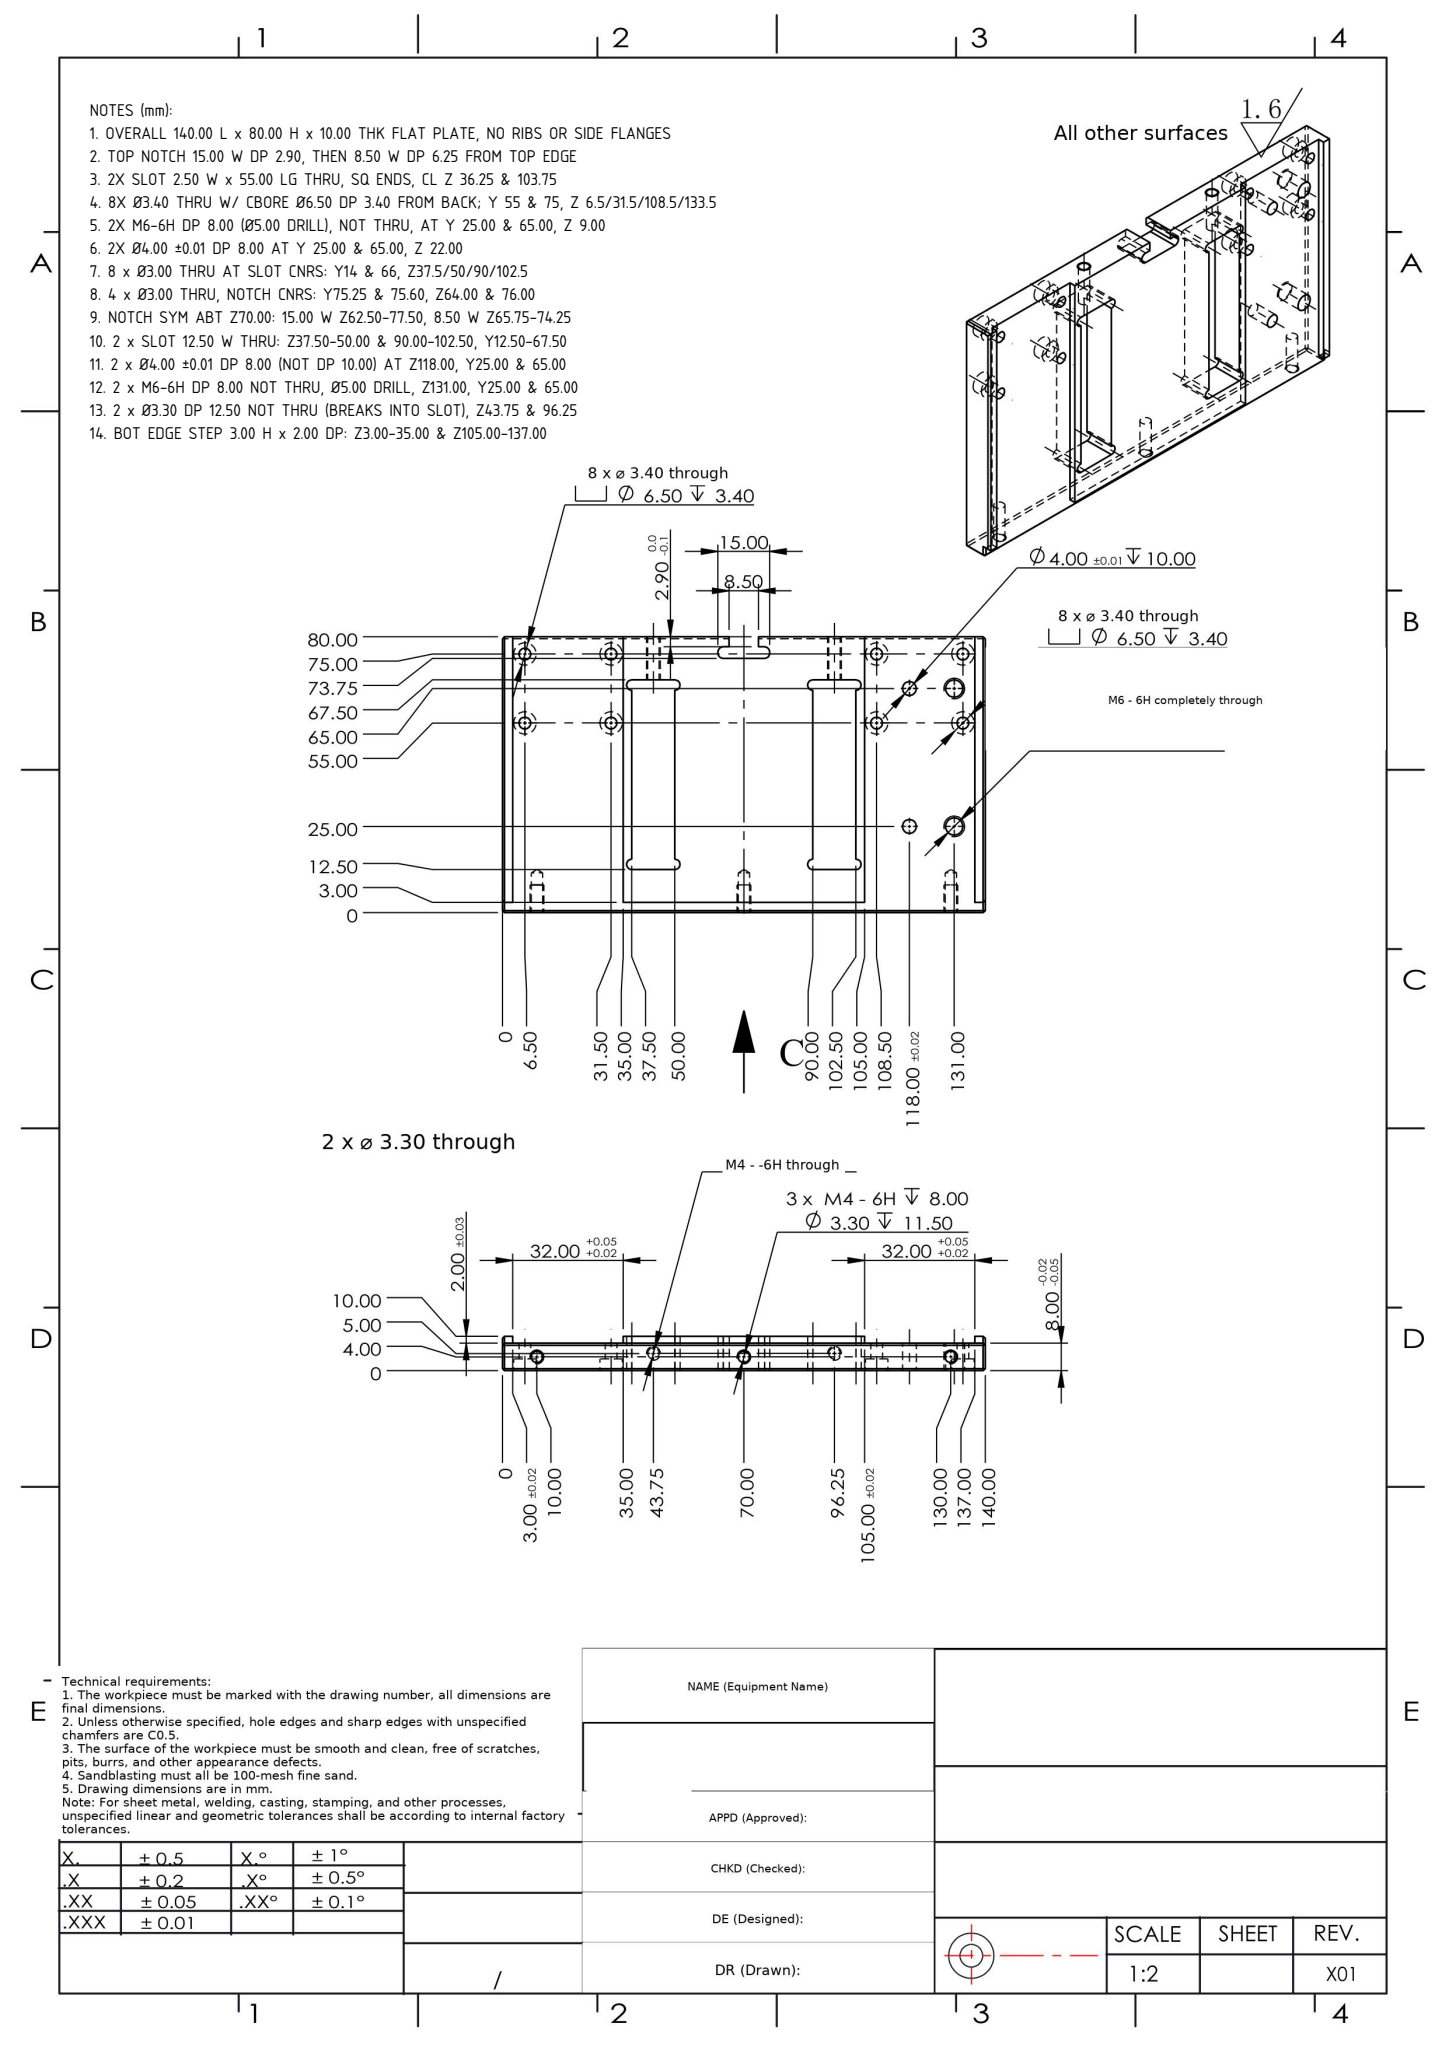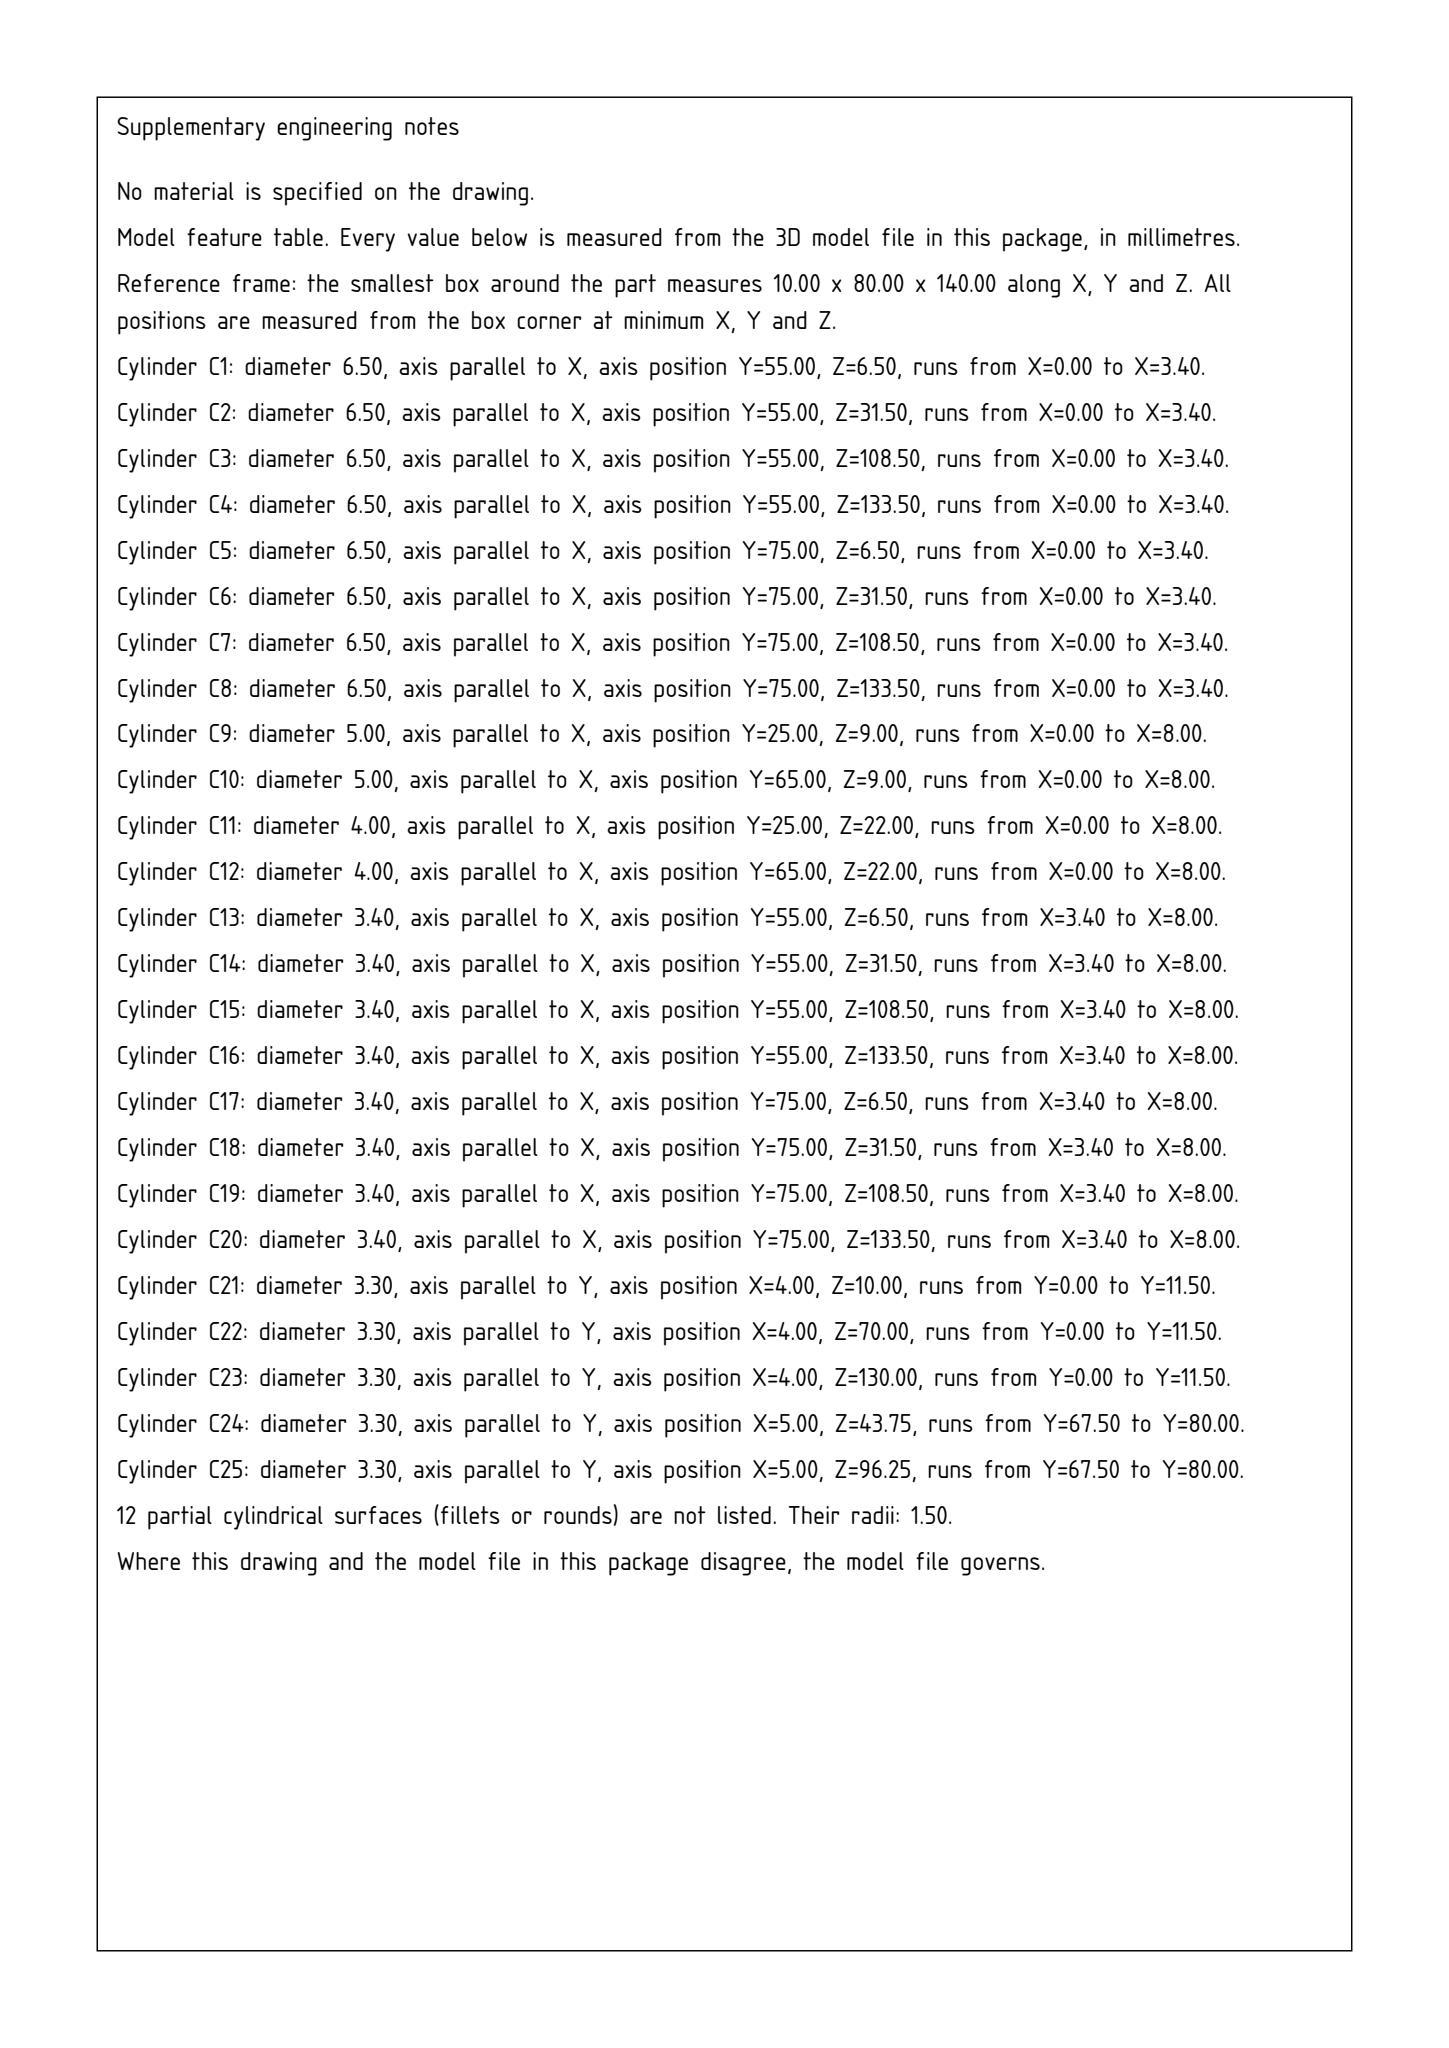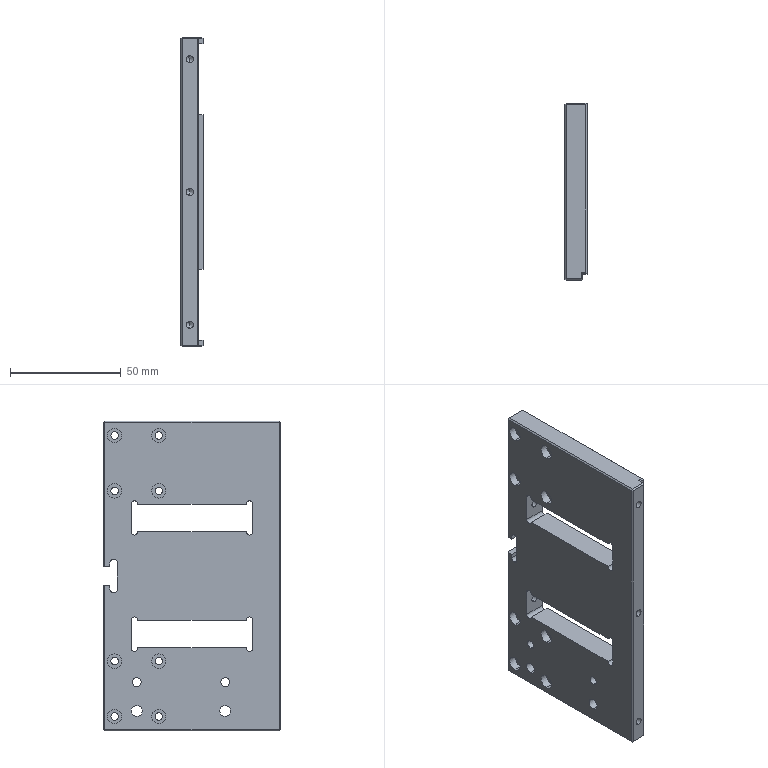Part | SolidWorks | mm | 1 solid | 134 faces | box 10 x 80 x 140 mm | volume 84134 mm3 | cylinder 66 | plane 62 | cone 6 | commonest cylinder face diameters 3 x16 6.5 x16 3.4 x16 3.3 x10 4 x4 5 x4
Drawing notes:
OVERALL 140.00 L x 80.00 H x 10.00 THK FLAT PLATE, NO RIBS OR SIDE FLANGES | from the solid: bbox_xyz = [10.0, 80.0, 140.0]; x planes only 0.0/3.4/8.0/10.0; z planes 0.0 & 140.0
TOP NOTCH 15.00 W DP 2.90, THEN 8.50 W DP 6.25 FROM TOP EDGE | from the solid: z 62.5/77.5 = 15.00; z 65.75/74.25 = 8.50; y 80.0-77.1 = 2.90; y 80.0-73.75 = 6.25
2X SLOT 2.50 W x 55.00 LG THRU, SQ ENDS, CL Z 36.25 & 103.75 | from the solid: z 35.0/37.5 and 102.5/105.0 = 2.50 W; y 12.5 & 67.5 = 55.00 LG; x 0.0/10.0 thru; no fillets
8X Ø3.40 THRU W/ CBORE Ø6.50 DP 3.40 FROM BACK; Y 55 & 75, Z 6.5/31.5/108.5/133.5 | from the solid: Ø3.4 & Ø6.5 x-axis cyls at y=55/75, z=6.5/31.5/108.5/133.5; x plane 3.4 = 8 CB bottoms
2X M6-6H DP 8.00 (Ø5.00 DRILL), NOT THRU, AT Y 25.00 & 65.00, Z 9.00 | from the solid: Ø5.0 x-axis cyls at (y25,z9) & (y65,z9), length 8.0; x plane at 8.0
2X Ø4.00 ±0.01 DP 8.00 AT Y 25.00 & 65.00, Z 22.00 | from the solid: Ø4.0 x-axis cyls at (y25,z22) & (y65,z22), length 8.0
8 x Ø3.00 THRU AT SLOT CNRS: Y14 & 66, Z37.5/50/90/102.5 | from the solid: Ø3.0 cyl, axis x, L=10.0 (thru 10 thk) at y=14.0 & 66.0, z=37.5, 50.0, 90.0, 102.5
4 x Ø3.00 THRU, NOTCH CNRS: Y75.25 & 75.60, Z64.00 & 76.00 | from the solid: Ø3.0 cyl, axis x, L=10.0 at (y75.25,z64), (y75.25,z76), (y75.6,z64), (y75.6,z76)
NOTCH SYM ABT Z70.00: 15.00 W Z62.50-77.50, 8.50 W Z65.75-74.25 | from the solid: z planes 62.5, 65.75, 74.25, 77.5; midpoint 70.0 = bbox z centre of 140
2 x SLOT 12.50 W THRU: Z37.50-50.00 & 90.00-102.50, Y12.50-67.50 | from the solid: z planes 37.5/50.0 & 90.0/102.5; y planes 12.5 (x2) & 67.5 (x2); dogbones 1.5 in from each
2 x Ø4.00 ±0.01 DP 8.00 (NOT DP 10.00) AT Z118.00, Y25.00 & 65.00 | from the solid: Ø4.0 cyl axis x, L=8.0 at y=25.0 & 65.0, z=22.0 from min cnr = 140-22 = 118.00 on dwg datum
2 x M6-6H DP 8.00 NOT THRU, Ø5.00 DRILL, Z131.00, Y25.00 & 65.00 | from the solid: Ø5.0 cyl axis x, L=8.0 at y=25.0 & 65.0, z=9.0 from min cnr = 140-9 = 131.00 on dwg datum
2 x Ø3.30 DP 12.50 NOT THRU (BREAKS INTO SLOT), Z43.75 & 96.25 | from the solid: Ø3.3 cyl axis y, L=12.5 from x=5.0 at z=43.75 & 96.25; slot top face y=67.5 = 80-12.5
BOT EDGE STEP 3.00 H x 2.00 DP: Z3.00-35.00 & Z105.00-137.00 | from the solid: y planes 0/3.0 (x3); x planes 10.0 & 8.0 = 2.00 dp; z breaks 3.0, 35.0, 105.0, 137.0
build123d program:
from build123d import *

# Parameters (mm, degrees)
SKETCH1_W                                       = 80
SKETCH1_H                                       = 140
BOSS_EXTRUDE1_DEPTH                             = 5
SKETCH6_W                                       = 32
SKETCH6_H                                       = 80
CUT_EXTRUDE5_DEPTH                              = 2
SKETCH7_W                                       = 12.5
SKETCH7_H                                       = 55
CUT_EXTRUDE6_DEPTH                              = 82.24
SKETCH8_W                                       = 140
SKETCH8_H                                       = 3
CUT_EXTRUDE7_DEPTH                              = 2
CUT_EXTRUDE8_DEPTH                              = 82.24
M3_HEX_SOCKET_HEAD_CAP_SCREW_CBORE1_D           = 3.4
M3_HEX_SOCKET_HEAD_CAP_SCREW_CBORE1_CBORE_D     = 6.5
M3_HEX_SOCKET_HEAD_CAP_SCREW_CBORE1_CBORE_DEPTH = 3.4
M4_TAPPED_HOLE1_D                               = 3.3
M4_TAPPED_HOLE1_DEPTH                           = 12.5
CHAMFER1_SIZE                                   = 0.6
M6_TAPPED_HOLE1_D                               = 5
HOLE1_D                                         = 4
HOLE2_D                                         = 3
FILLET1_R                                       = 1.5
M4_TAPPED_HOLE2_D                               = 3.3
M4_TAPPED_HOLE2_DEPTH                           = 11.5
M4_TAPPED_HOLE2_TIP                             = 0.9914


with BuildPart() as part:
    # Sketch1 → Boss-Extrude1 (new, symmetric)
    with BuildSketch(Plane(origin=(0, 0, 0), x_dir=(0, -1, 0), z_dir=(1, 0, 0))):
        Rectangle(SKETCH1_W, SKETCH1_H)
    extrude(amount=BOSS_EXTRUDE1_DEPTH, both=True)

    # Sketch6 → Cut-Extrude5 (cut)
    with BuildSketch(Plane(origin=(5, 0, 0), x_dir=(0, 0, -1), z_dir=(1, 0, 0))):
        with Locations((51, 0)):
            Rectangle(SKETCH6_W, SKETCH6_H)
        with Locations((-51, 0)):
            Rectangle(SKETCH6_W, SKETCH6_H)
    extrude(amount=-CUT_EXTRUDE5_DEPTH, mode=Mode.SUBTRACT)

    # Sketch7 → Cut-Extrude6 (cut, through all)
    with BuildSketch(Plane(origin=(5, 0, 0), x_dir=(0, 0, -1), z_dir=(1, 0, 0))):
        with Locations((26.25, 0)):
            Rectangle(SKETCH7_W, SKETCH7_H)
        with Locations((-26.25, 0)):
            Rectangle(SKETCH7_W, SKETCH7_H)
    extrude(amount=-CUT_EXTRUDE6_DEPTH, mode=Mode.SUBTRACT)

    # Sketch8 → Cut-Extrude7 (cut)
    with BuildSketch(Plane(origin=(5, 0, 0), x_dir=(0, 0, -1), z_dir=(1, 0, 0))):
        with Locations((0, -38.5)):
            Rectangle(SKETCH8_W, SKETCH8_H)
    extrude(amount=-CUT_EXTRUDE7_DEPTH, mode=Mode.SUBTRACT)

    # Sketch9 → Cut-Extrude8 (cut, through all)
    with BuildSketch(Plane(origin=(5, 0, 0), x_dir=(0, 0, -1), z_dir=(1, 0, 0))):
        Polygon((-4.25, 40), (-4.25, 37.1), (-7.5, 37.1), (-7.5, 33.75), (7.5, 33.75), (7.5, 37.1), (4.25, 37.1), (4.25, 40), align=None)
    extrude(amount=-CUT_EXTRUDE8_DEPTH, mode=Mode.SUBTRACT)

    # M3 Hex Socket Head Cap Screw CBORE1 (through all)
    with Locations(Plane.ZY.offset(5)):
        with Locations((-63.5, 15), (-63.5, 35), (-38.5, 15), (-38.5, 35), (38.5, 15), (38.5, 35), (63.5, 15), (63.5, 35)):
            CounterBoreHole(M3_HEX_SOCKET_HEAD_CAP_SCREW_CBORE1_D / 2, M3_HEX_SOCKET_HEAD_CAP_SCREW_CBORE1_CBORE_D / 2, M3_HEX_SOCKET_HEAD_CAP_SCREW_CBORE1_CBORE_DEPTH)

    # M4 Tapped Hole1
    with Locations(Plane(origin=(0, 40, 0), x_dir=(1, 0, 0), z_dir=(0, 1, 0))):
        with Locations((0, 26.25), (0, -26.25)):
            Hole(M4_TAPPED_HOLE1_D / 2, depth=M4_TAPPED_HOLE1_DEPTH)

    # Chamfer1
    chamfer1_edges = [part.edges().sort_by_distance(p)[0] for p in [
        (-5, 40, 37.125),
        (3, -40, 0),
        (-5, 0, -70),
        (-5, -40, 0),
        (-5, 0, 70),
        (-5, 40, -37.125),
        (5, 1.5, 70),
        (0, 40, -70),
        (0, 40, 70),
        (5, 1.5, -70),
        (-1, -40, -70),
        (-1, -40, 70),
        (3, -38.5, -70),
        (3, -38.5, 70),
        (4, -37, 70),
        (4, -37, -70),
    ]]
    chamfer(chamfer1_edges, length=CHAMFER1_SIZE)

    # M6 Tapped Hole1 (through all)
    with Locations(Plane.ZY.offset(5)):
        with Locations((-61, -15), (-61, 25)):
            Hole(M6_TAPPED_HOLE1_D / 2)

    # Hole1 (through all)
    with Locations(Plane.ZY.offset(5)):
        with Locations((-48, -15), (-48, 25)):
            Hole(HOLE1_D / 2)

    # Hole2 (through all)
    with Locations(Plane.ZY.offset(5)):
        with Locations((32.5, -26), (20, -26), (32.5, 26), (20, 26), (-20, -26), (-32.5, -26), (-20, 26), (-32.5, 26)):
            Hole(HOLE2_D / 2)

    # Fillet1
    fillet1_edges = [part.edges().sort_by_distance(p)[0] for p in [
        (0, 37.1, -7.5),
        (0, 33.75, -7.5),
        (0, 33.75, 7.5),
        (0, 37.1, 7.5),
    ]]
    fillet(fillet1_edges, radius=FILLET1_R)

    # M4 Tapped Hole2
    with Locations(Plane(origin=(0, -40, 0), x_dir=(-1, 0, 0), z_dir=(0, -1, 0))):
        with Locations((1, -60), (1, 0), (1, 60)):
            Hole(M4_TAPPED_HOLE2_D / 2, depth=M4_TAPPED_HOLE2_DEPTH)
            with Locations((0, 0, -(M4_TAPPED_HOLE2_DEPTH + M4_TAPPED_HOLE2_TIP / 2))):  # 118° drill point
                Cone(0, M4_TAPPED_HOLE2_D / 2, M4_TAPPED_HOLE2_TIP, mode=Mode.SUBTRACT)


solid = part.part